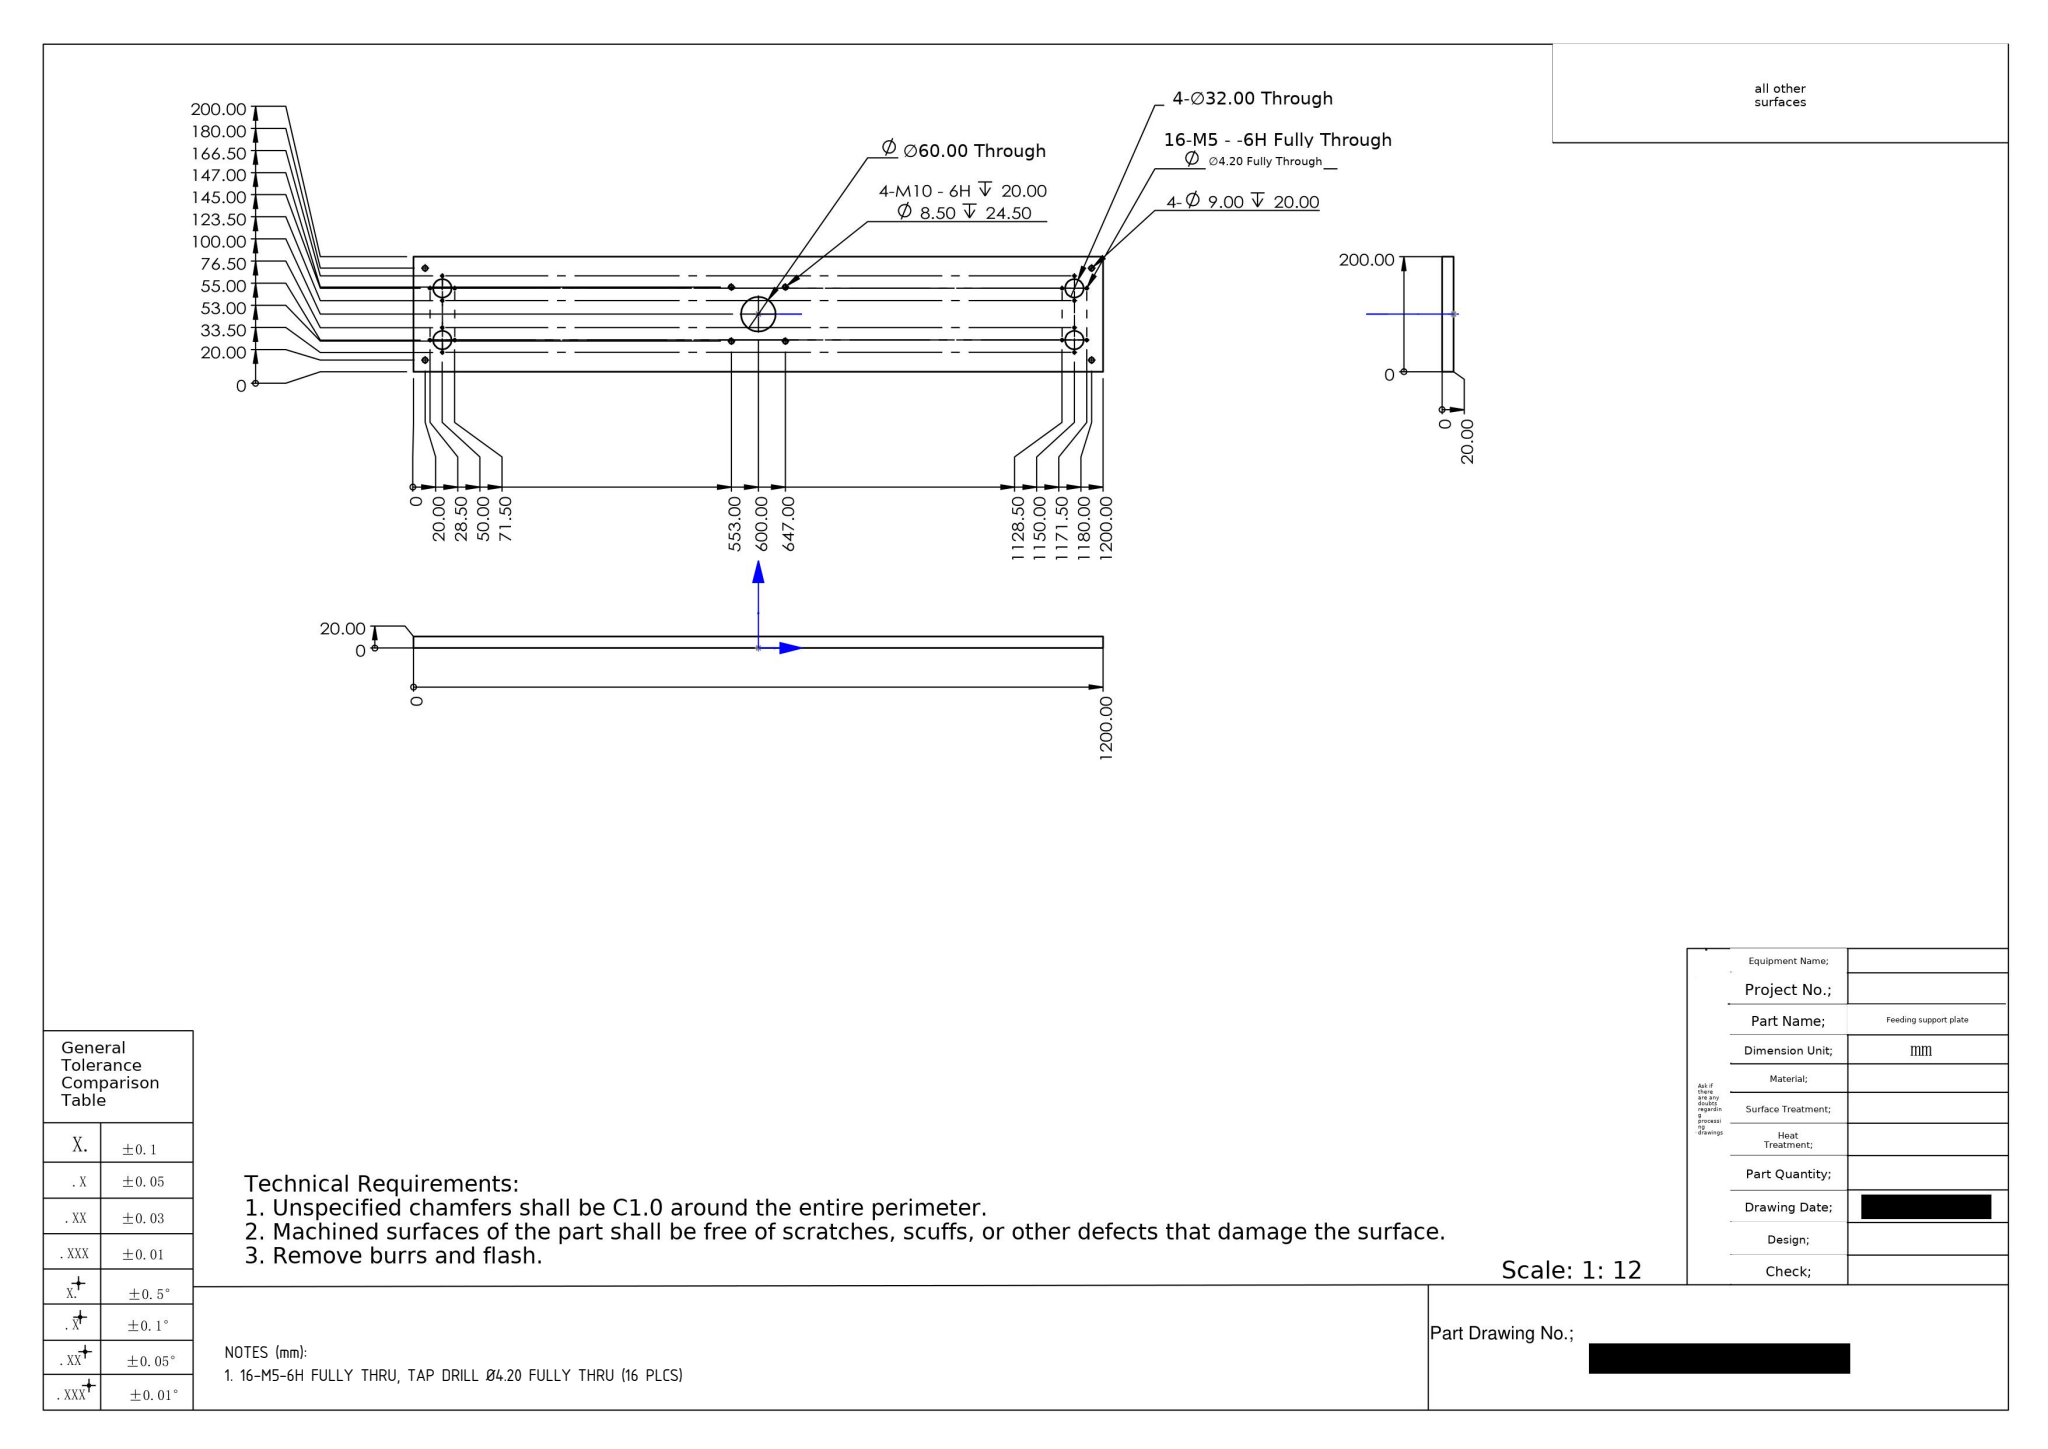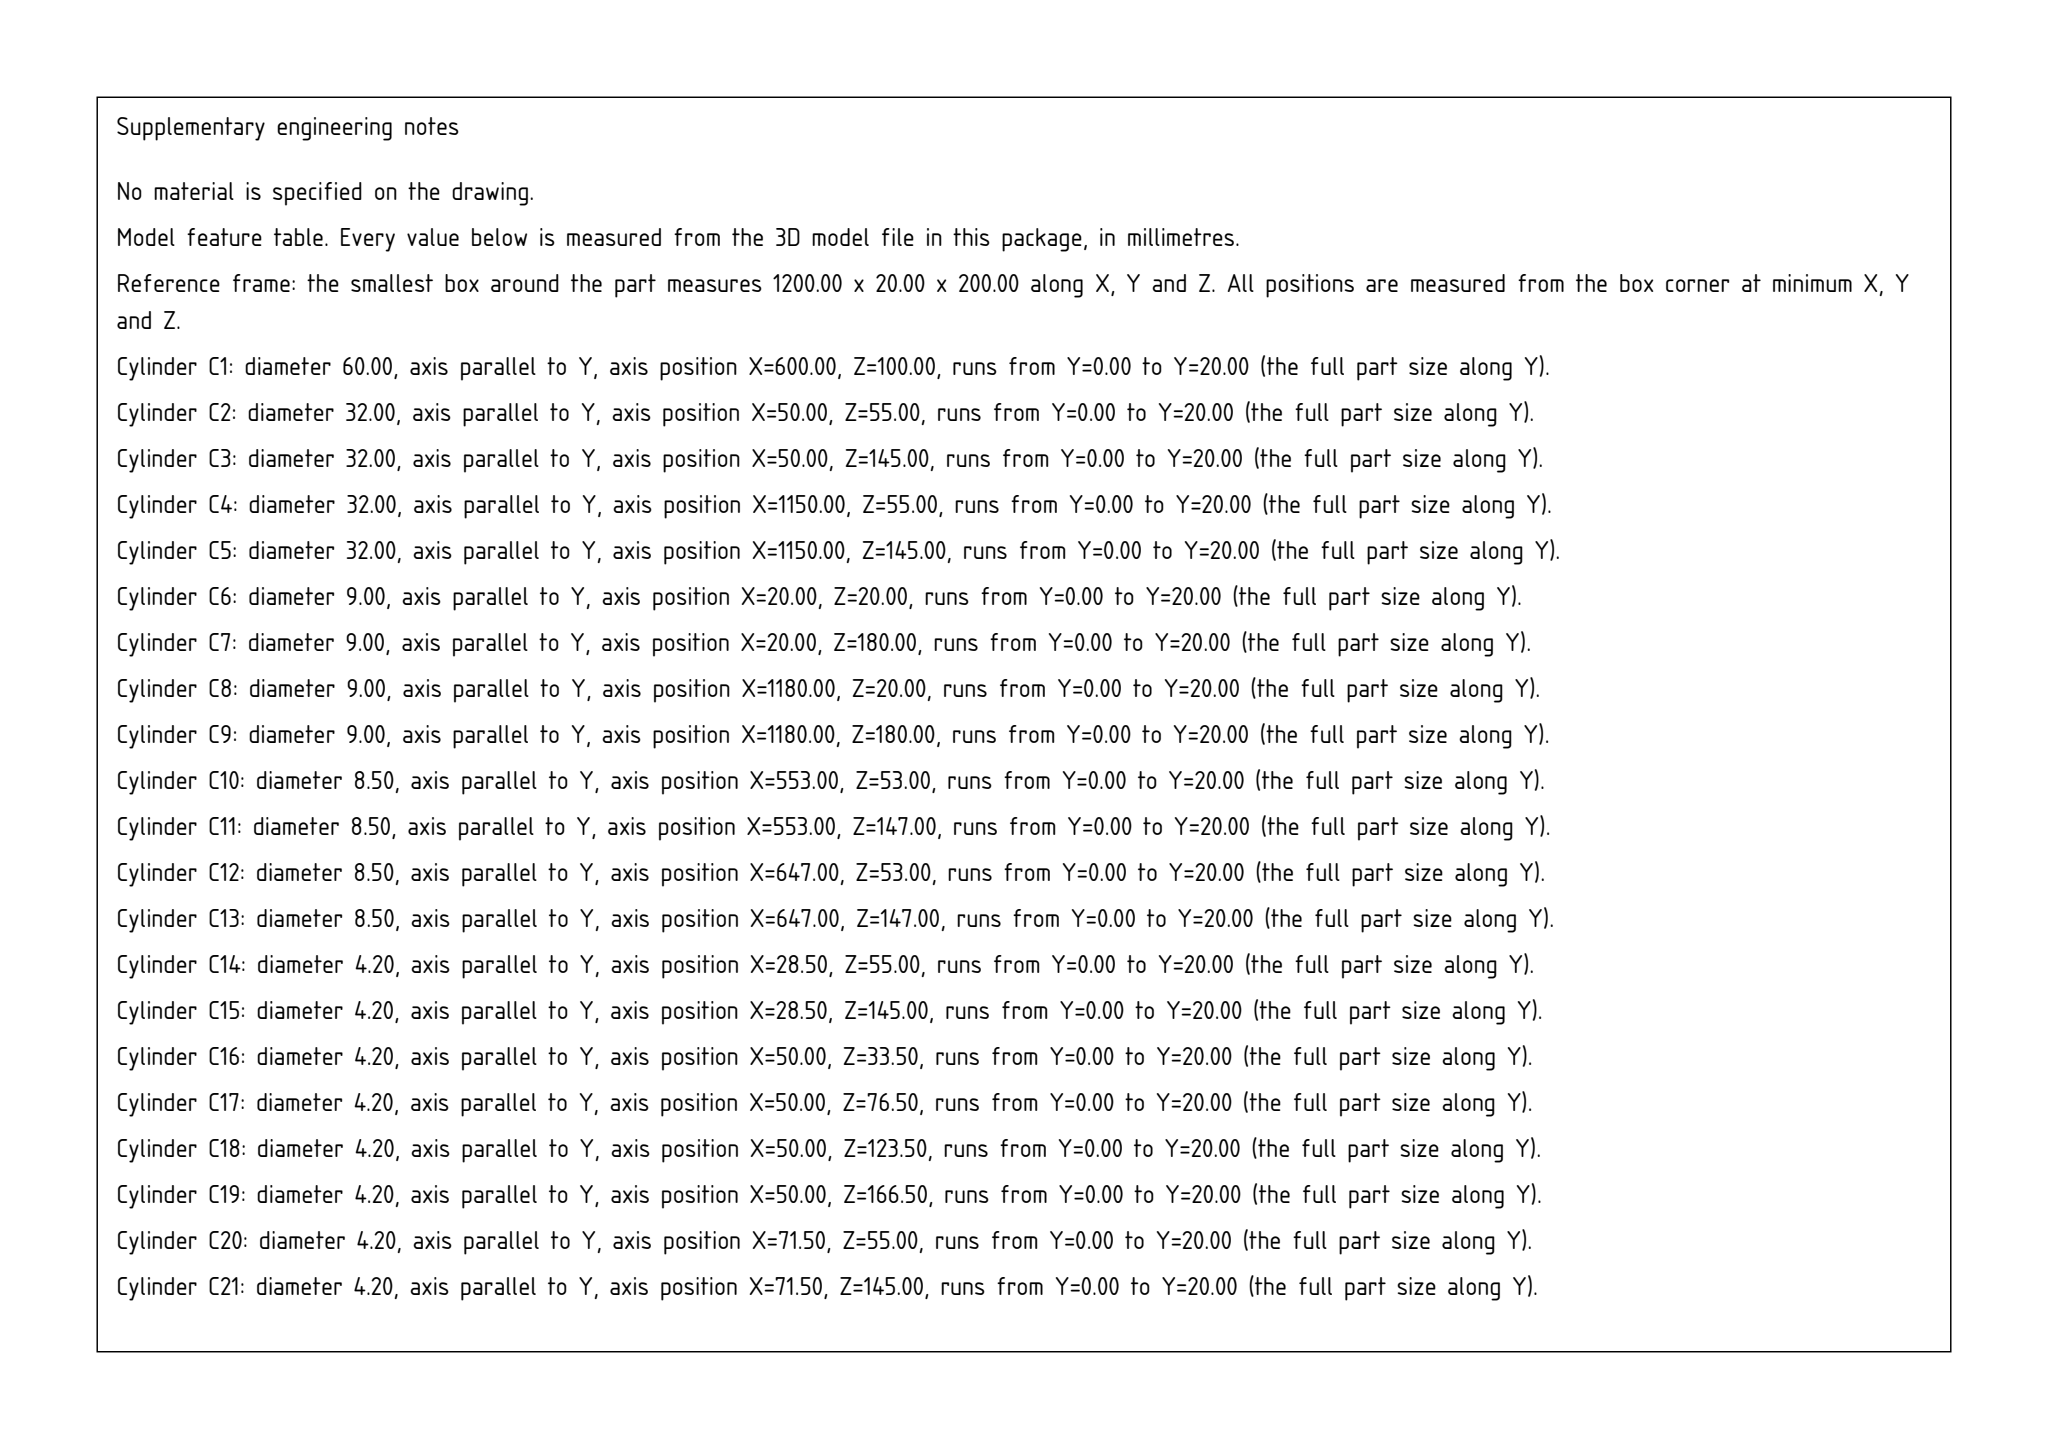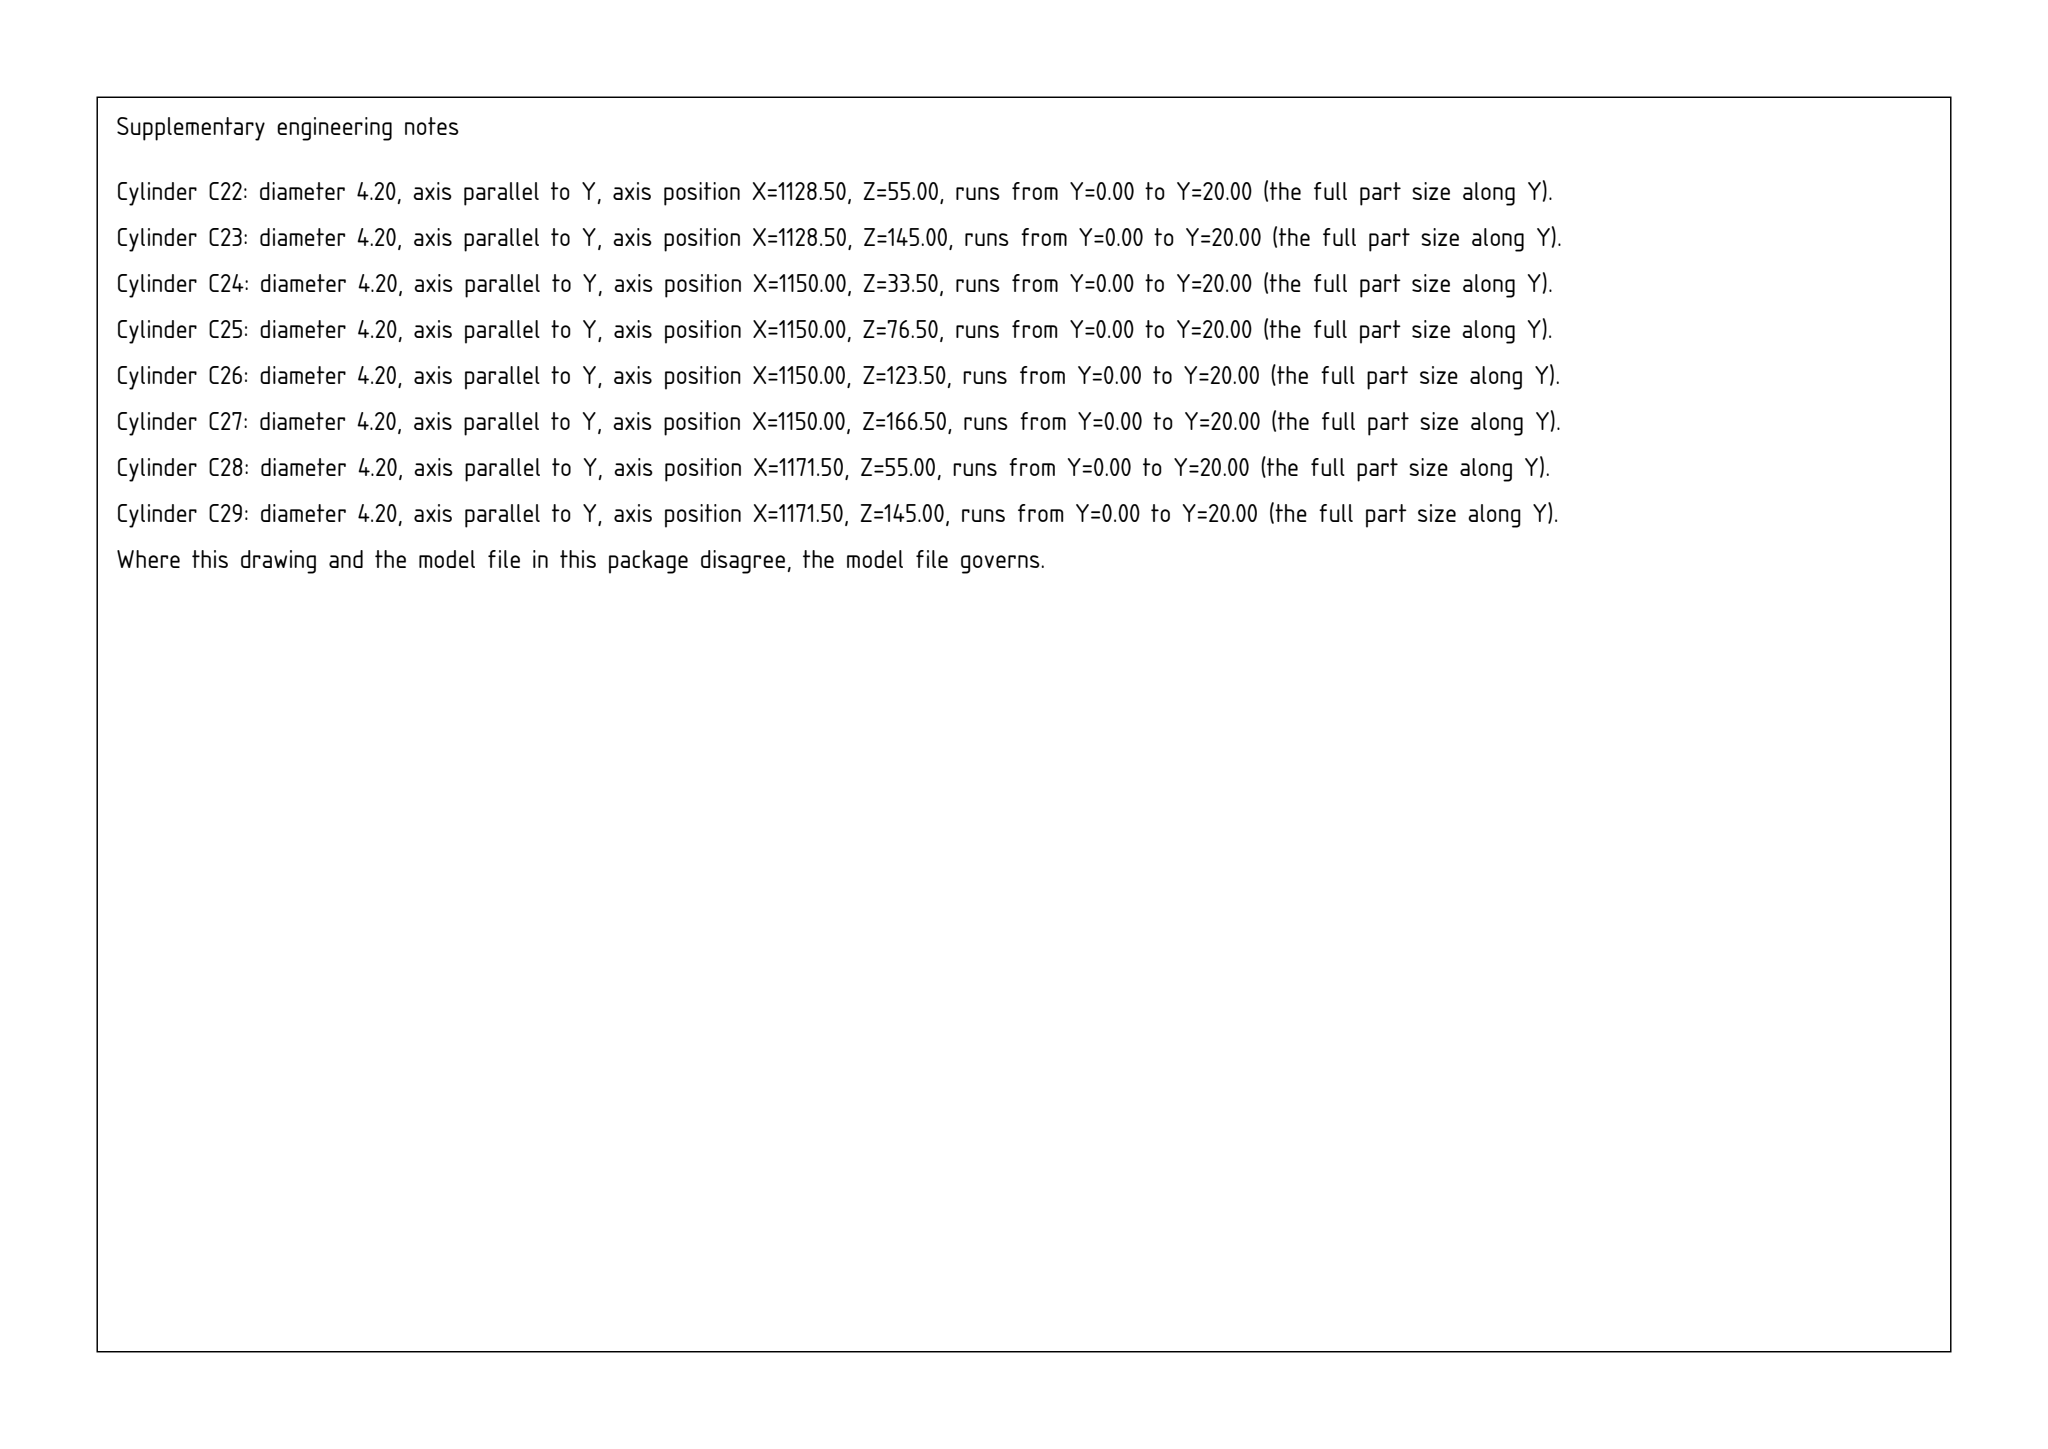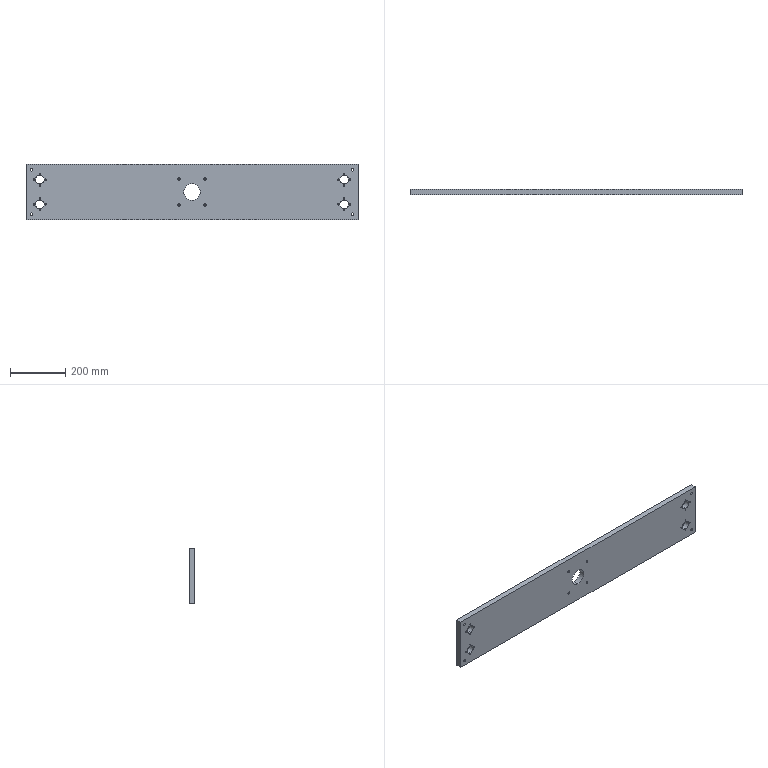Part | SolidWorks | mm | 1 solid | 64 faces | box 1200 x 20 x 200 mm | volume 4665049 mm3 | cylinder 58 | plane 6 | commonest cylinder face diameters 4.2 x32 32 x8 8.5 x8 9 x8 60 x2
Drawing notes:
16-M5-6H FULLY THRU, TAP DRILL Ø4.20 FULLY THRU (16 PLCS) | from the solid: 16 cylinders dia 4.20, axis y, length 20.0 (full 20 thk) at x=28.5/50/71.5/1128.5/1150/1171.5, z=33.5/55/76.5/123.5/145/166.5
build123d program:
from build123d import *

# Parameters (mm, degrees)
SKETCH1_W                = 1200
SKETCH1_H                = 200
BOSS_EXTRUDE1_DEPTH      = 20
M8_CLEARANCE_HOLE1_D     = 9
M8_CLEARANCE_HOLE1_DEPTH = 20
M8_CLEARANCE_HOLE1_TIP   = 2.704
M10_TAPPED_HOLE1_D       = 8.5
M10_TAPPED_HOLE1_DEPTH   = 24.5
M10_TAPPED_HOLE1_TIP     = 2.554
SKETCH8_R                = 30
CUT_EXTRUDE1_DEPTH       = 609.605
SKETCH9_R                = 16
CUT_EXTRUDE2_DEPTH       = 609.605
M5_TAPPED_HOLE1_D        = 4.2
LPATTERN1_COUNT          = 2
LPATTERN1_PITCH          = 1100
LPATTERN1_COUNT_DIR2     = 2
LPATTERN1_PITCH_DIR2     = 90


with BuildPart() as part:
    # Sketch1 → Boss-Extrude1 (new body)
    with BuildSketch(Plane(origin=(0, 0, 0), x_dir=(1, 0, 0), z_dir=(0, 1, 0))):
        Rectangle(SKETCH1_W, SKETCH1_H)
    extrude(amount=BOSS_EXTRUDE1_DEPTH)

    # M8 Clearance Hole1
    with Locations(Plane(origin=(0, 0, 0), x_dir=(-1, 0, 0), z_dir=(0, -1, 0))):
        with Locations((-580, 80), (-580, -80), (580, -80), (580, 80)):
            Hole(M8_CLEARANCE_HOLE1_D / 2, depth=M8_CLEARANCE_HOLE1_DEPTH)
            with Locations((0, 0, -(M8_CLEARANCE_HOLE1_DEPTH + M8_CLEARANCE_HOLE1_TIP / 2))):  # 118° drill point
                Cone(0, M8_CLEARANCE_HOLE1_D / 2, M8_CLEARANCE_HOLE1_TIP, mode=Mode.SUBTRACT)

    # M10 Tapped Hole1
    with Locations(Plane(origin=(0, 20, 0), x_dir=(1, 0, 0), z_dir=(0, 1, 0))):
        with Locations((-47, 47), (47, 47), (-47, -47), (47, -47)):
            Hole(M10_TAPPED_HOLE1_D / 2, depth=M10_TAPPED_HOLE1_DEPTH)
            with Locations((0, 0, -(M10_TAPPED_HOLE1_DEPTH + M10_TAPPED_HOLE1_TIP / 2))):  # 118° drill point
                Cone(0, M10_TAPPED_HOLE1_D / 2, M10_TAPPED_HOLE1_TIP, mode=Mode.SUBTRACT)

    # Sketch8 → Cut-Extrude1 (cut, through all)
    with BuildSketch(Plane(origin=(0, 20, 0), x_dir=(1, 0, 0), z_dir=(0, 1, 0))):
        with Locations(Location((0, 0, 0), (0, 0, 270))):
            Circle(SKETCH8_R)
    extrude(amount=-CUT_EXTRUDE1_DEPTH, mode=Mode.SUBTRACT)

    # Sketch9 → Cut-Extrude2 (cut, through all)
    with BuildSketch(Plane(origin=(0, 20, 0), x_dir=(1, 0, 0), z_dir=(0, 1, 0))):
        with Locations(Location((-550, 45, 0), (0, 0, 270))):
            Circle(SKETCH9_R)
        with Locations(Location((-550, -45, 0), (0, 0, 270))):
            Circle(SKETCH9_R)
        with Locations(Location((550, 45, 0), (0, 0, 270))):
            Circle(SKETCH9_R)
        with Locations(Location((550, -45, 0), (0, 0, 270))):
            Circle(SKETCH9_R)
    extrude(amount=-CUT_EXTRUDE2_DEPTH, mode=Mode.SUBTRACT)

    # M5 Tapped Hole1 (through all)
    with Locations(Plane(origin=(0, 20, 0), x_dir=(1, 0, 0), z_dir=(0, 1, 0))):
        with Locations((-550, 23.5), (-550, 66.5), (-571.5, 45), (-528.5, 45)):
            m5_tapped_hole1 = Hole(M5_TAPPED_HOLE1_D / 2)

    # LPattern1: M5 Tapped Hole1 2 × 2
    with Locations(*[(i * LPATTERN1_PITCH, 0, j * LPATTERN1_PITCH_DIR2) for i in range(LPATTERN1_COUNT) for j in range(LPATTERN1_COUNT_DIR2) if (i, j) != (0, 0)]):
        add(m5_tapped_hole1, mode=Mode.SUBTRACT)


solid = part.part